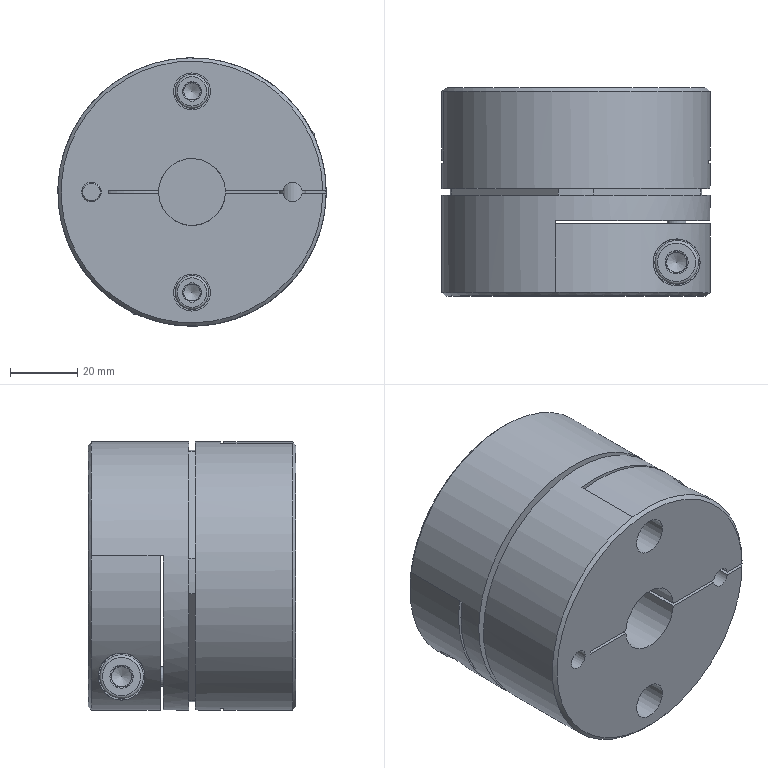Assembly | NX | mm | 13 component files | 13 solids | 258 faces | box 80 x 62 x 80 mm | volume 267060 mm3 | plane 132 | cylinder 64 | cone 50 | torus 12 | commonest cylinder face diameters 5.795 x16 6.6 x8 10 x8 11 x8 75 x4 80 x4 20 x4 7.76 x4
Bill of materials:
unnamed part 1 | 1 |  | Thin flat square plate with its four corners cut back by circular arcs, and four round through-holes, one near each corner.
GB-T70.1-2000,M8x25 | 2 |  | Hexagon Socket Head Cap Screw, GB-T 70.1-2000,M8x25
unnamed part 2 | 2 |  | Thick cylindrical disc/hub with a central through-bore, four axial holes on two perpendicular axes (two larger, two smaller), and a narrow slit cut in from the outside edge partway through the thickness, crossed by a hole through the side; looks like a split clamping hub.
GB-T70.1-2000,M6x12 | 4 |  | Hexagon Socket Head Cap Screw, GB-T 70.1-2000,M6x12
unnamed part 3 | 4 |  | Plain flat annular ring (washer-like) with a rectangular cross-section, round concentric outer and inner edges, and constant thickness.
Mates:
1. concentric | Half_Diaphragm_Coupling 2 edge | Diaphragm 1 edge
2. fix | Diaphragm 1 component
3. concentric | Half_Diaphragm_Coupling 1 edge | Diaphragm 1 edge
4. concentric | Washer_6 4 edge | Diaphragm 1 edge
5. bond | Half_Diaphragm_Coupling 2 component | assembly component
6. bond | Washer_6 4 component | assembly component
7. bond | Washer_6 3 component | assembly component
8. circular | assembly datumaxis | assembly cartesiancoordinatesystem | assembly cartesiancoordinatesystem
9. bond | GB-T70_1-2000_M6x12 4 component | assembly component
10. bond | GB-T70_1-2000_M6x12 3 component | assembly component
11. circular | assembly datumaxis | assembly cartesiancoordinatesystem | assembly cartesiancoordinatesystem
12. concentric | Washer_6 2 edge | Diaphragm 1 edge
13. bond | GB-T70_1-2000_M6x12 2 component | assembly component
14. bond | GB-T70_1-2000_M6x12 1 component | assembly component
15. circular | assembly datumaxis | assembly cartesiancoordinatesystem | assembly cartesiancoordinatesystem
16. bond | Washer_6 2 component | assembly component
17. bond | Washer_6 1 component | assembly component
18. circular | assembly datumaxis | assembly cartesiancoordinatesystem | assembly cartesiancoordinatesystem